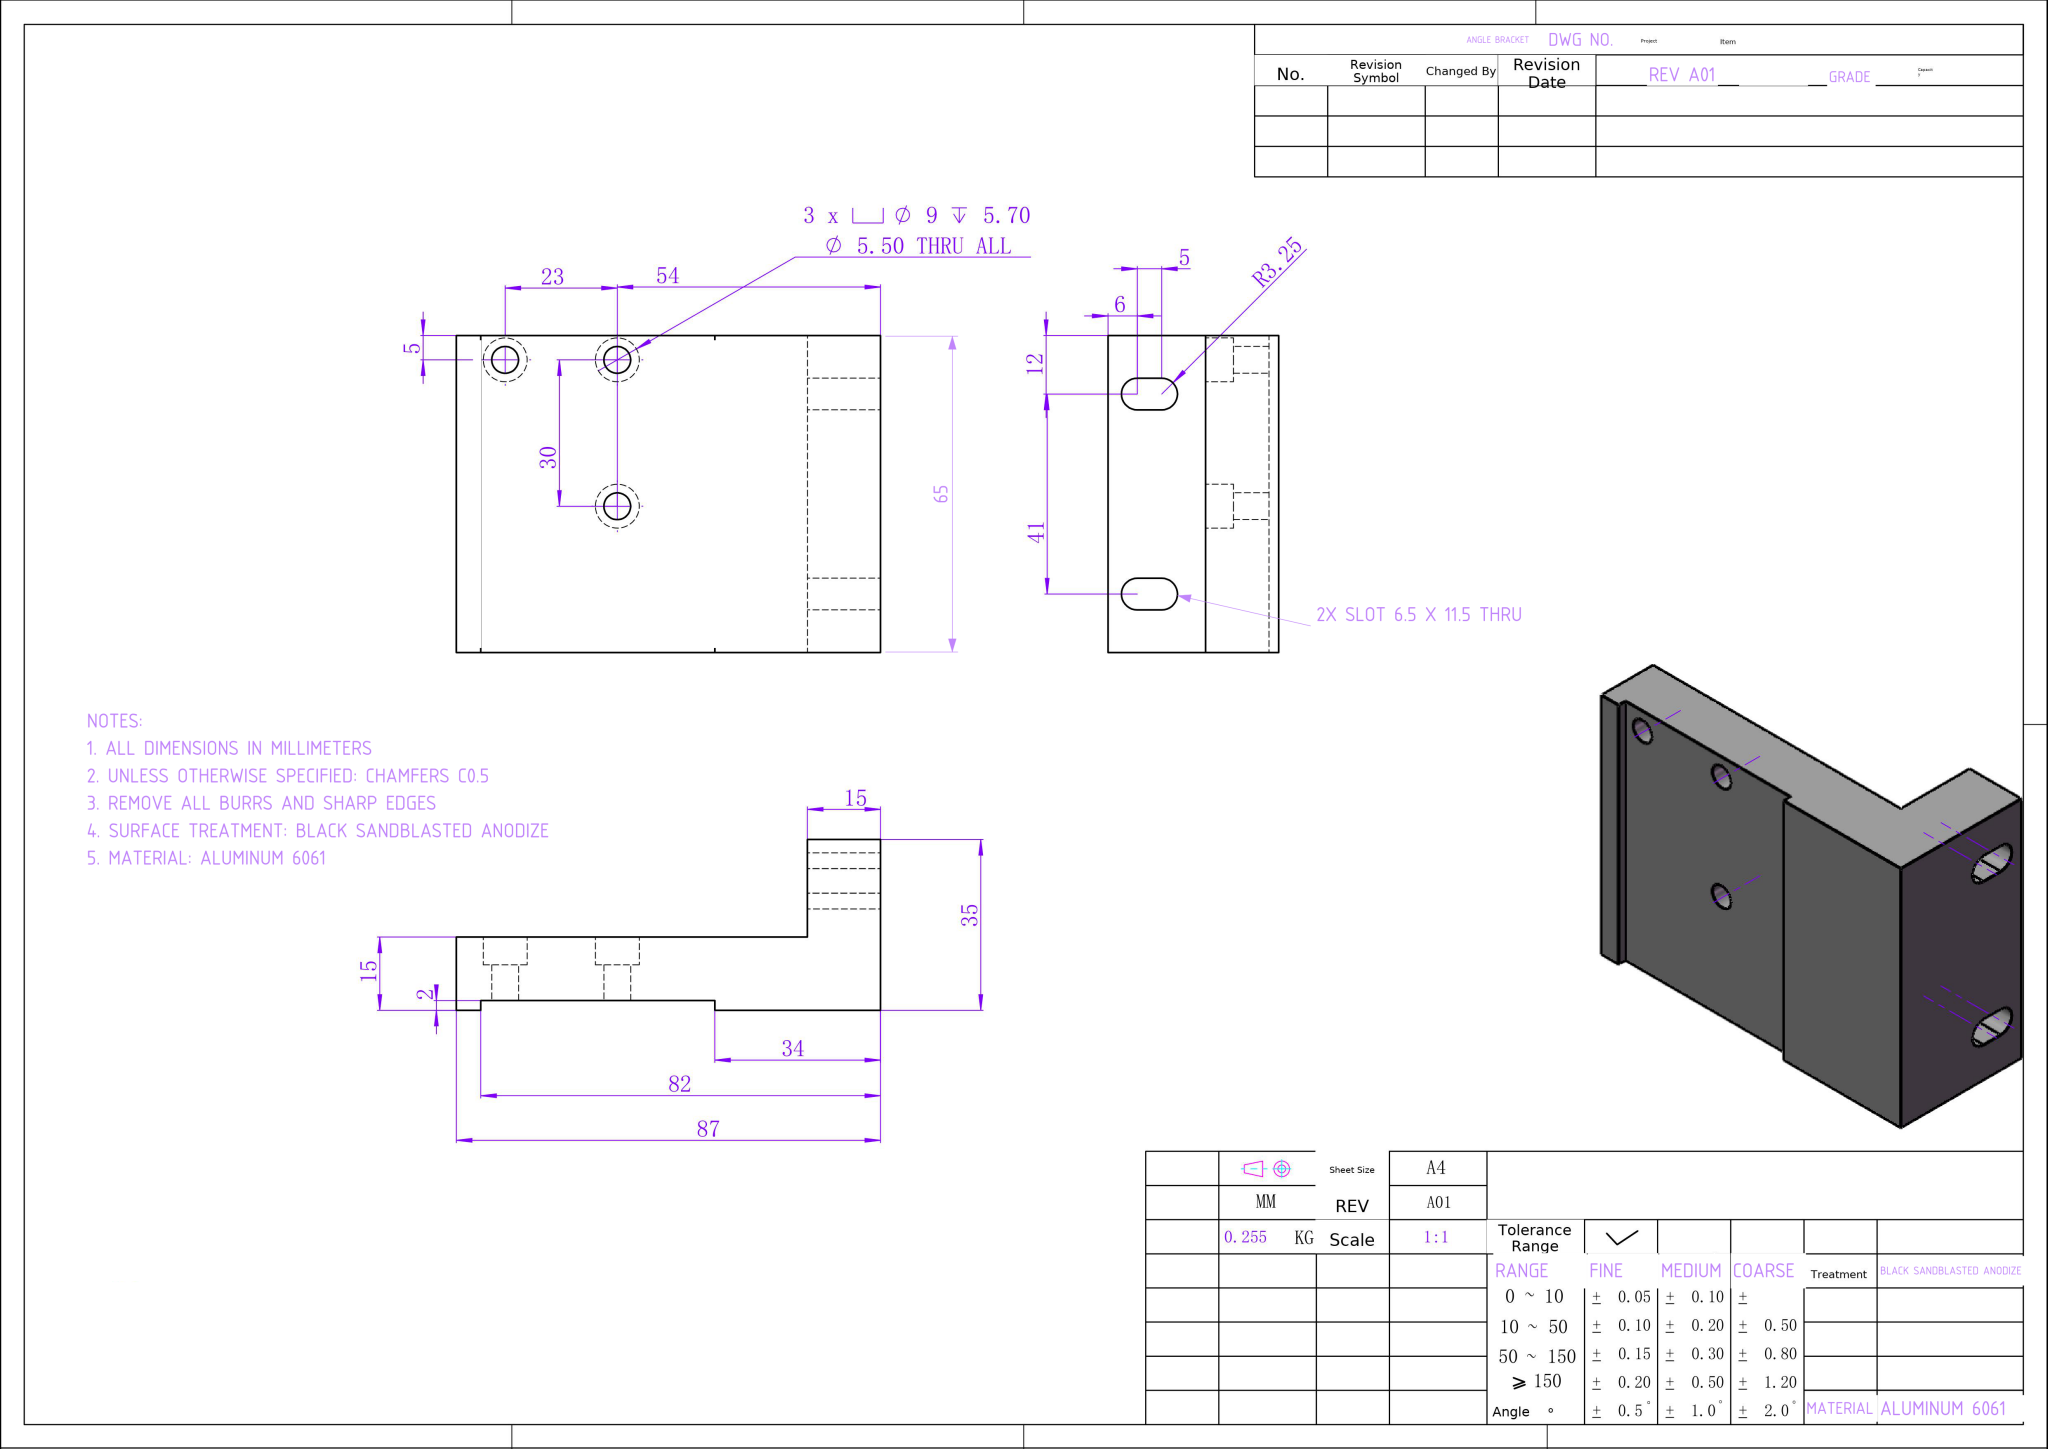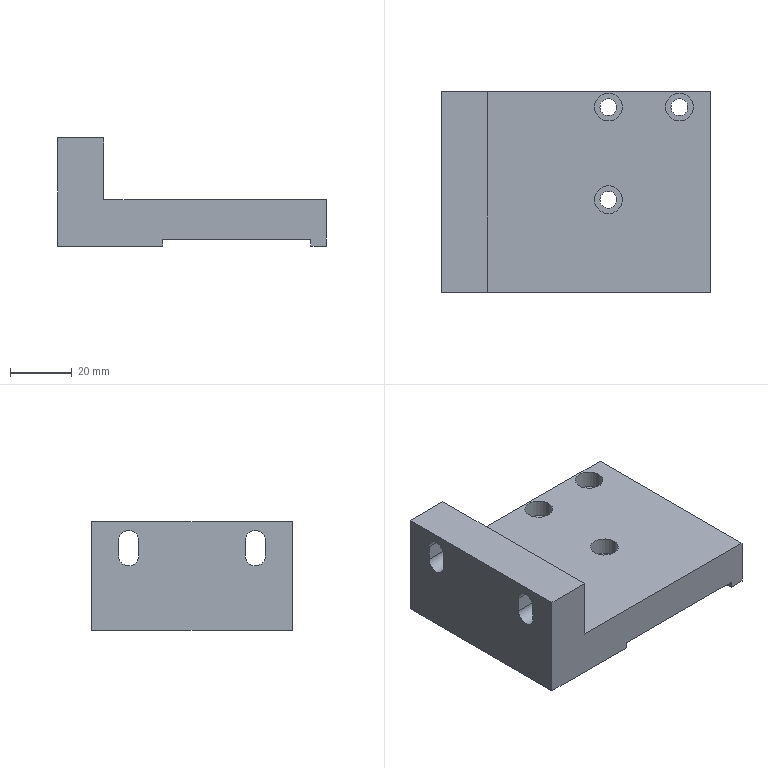Part | NX | mm | 1 solid | 35 faces | box 87 x 65 x 35 mm | volume 94506 mm3 | plane 19 | cylinder 16 | commonest cylinder face diameters 5.5 x6 9 x6 6.5 x4